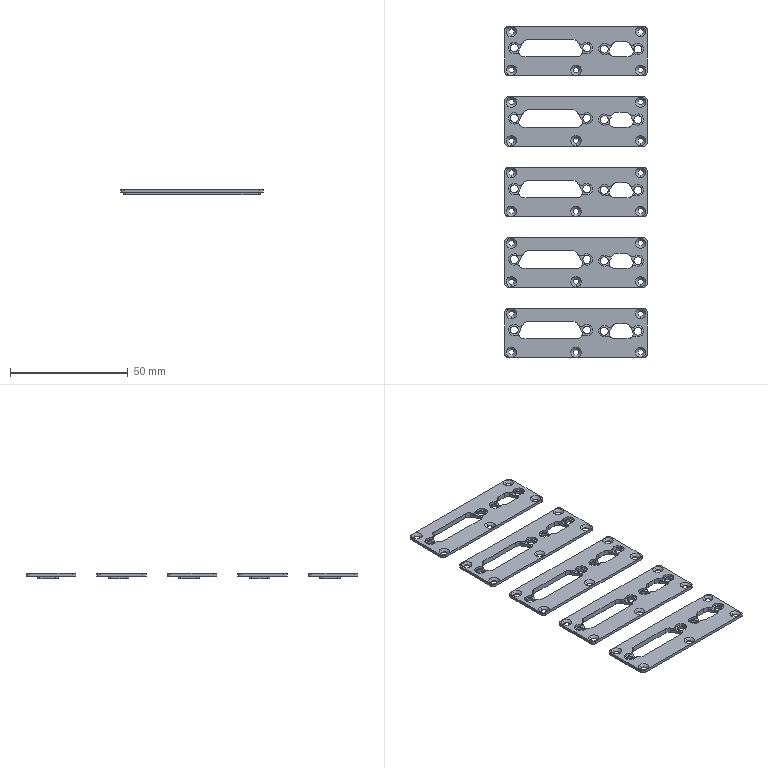CAM job | Mastercam | mm | 16 operations | part box 60.5 x 141 x 2.2
1. 2D High Speed (2D Area Mill) | 3 - 3 平铣刀
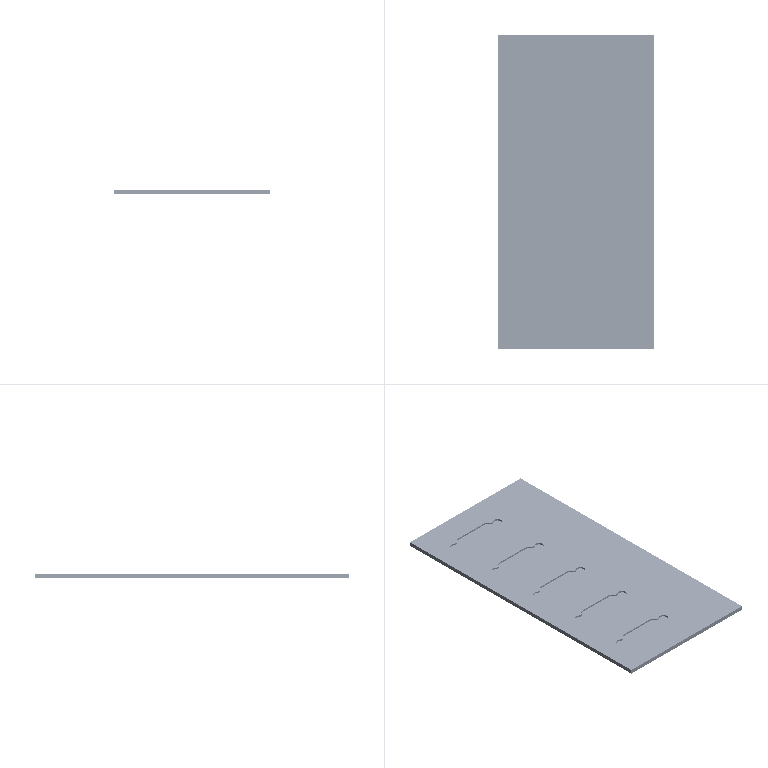2. 2D High Speed (2D Area Mill) | 3 - 3 平铣刀
3. Contour (Ramp) | 3 - 3 平铣刀
4. Contour (Ramp) | 3 - 3 平铣刀
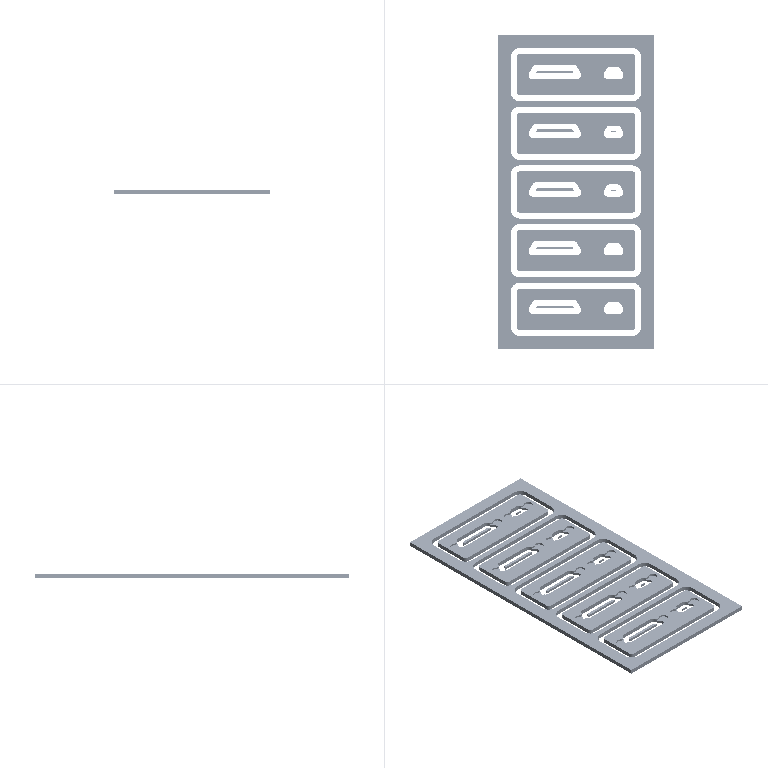5. Contour (2D chamfer) | 7 - 4 倒角刀
6. 2D High Speed (2D Area Mill) | 2 - 2 平铣刀
7. 2D High Speed (2D Area Mill) | 2 - 2 平铣刀
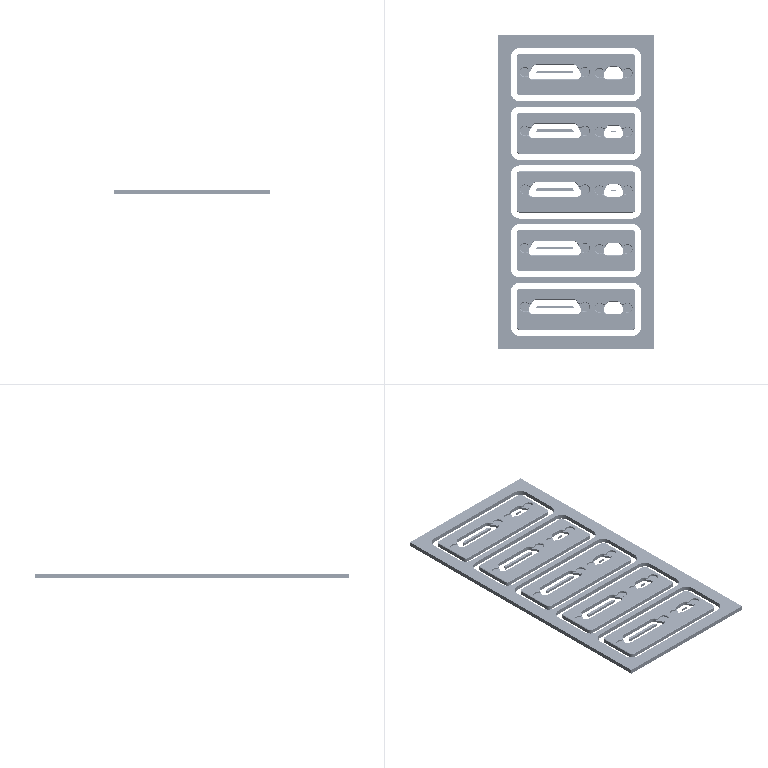8. Contour (2D) | 2 - 2 平铣刀
9. Contour (2D) | 2 - 2 平铣刀
10. Contour (2D) | 2 - 2 平铣刀
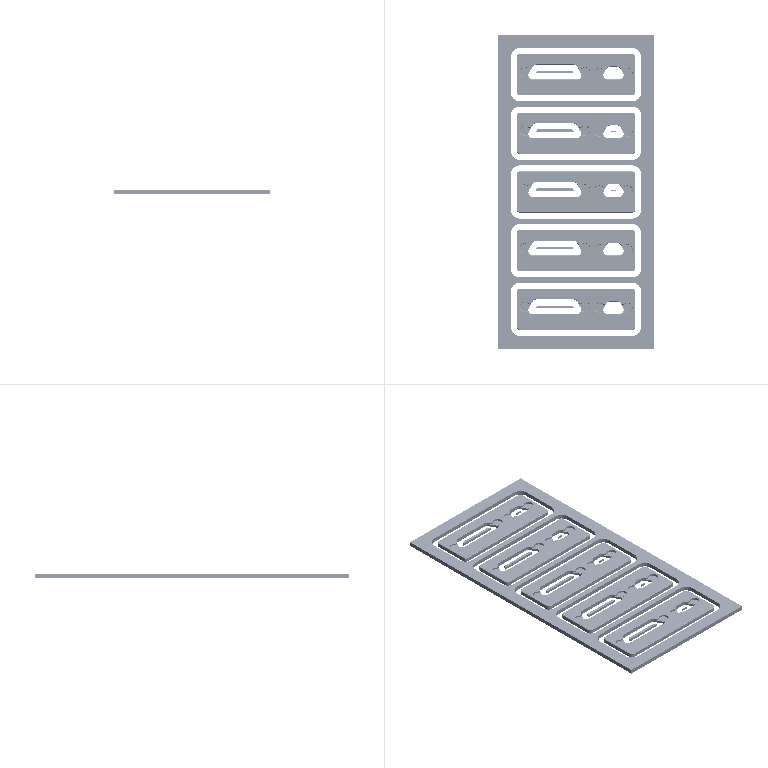11. Contour (2D) | 2 - 2 平铣刀
12. Facing | 6 - 6 平铣刀
13. Contour (Ramp) | 6 - 6 平铣刀
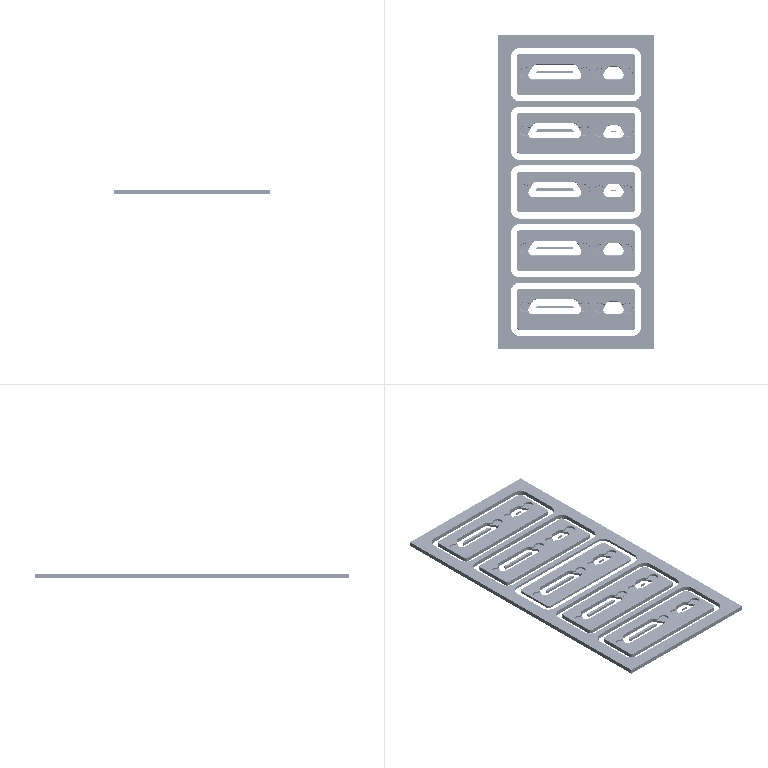14. Contour (2D) | 6 - 6 平铣刀
15. Contour (2D chamfer) | 7 - 4 倒角刀
16. Drill/Counterbore | 7 - 4 倒角刀